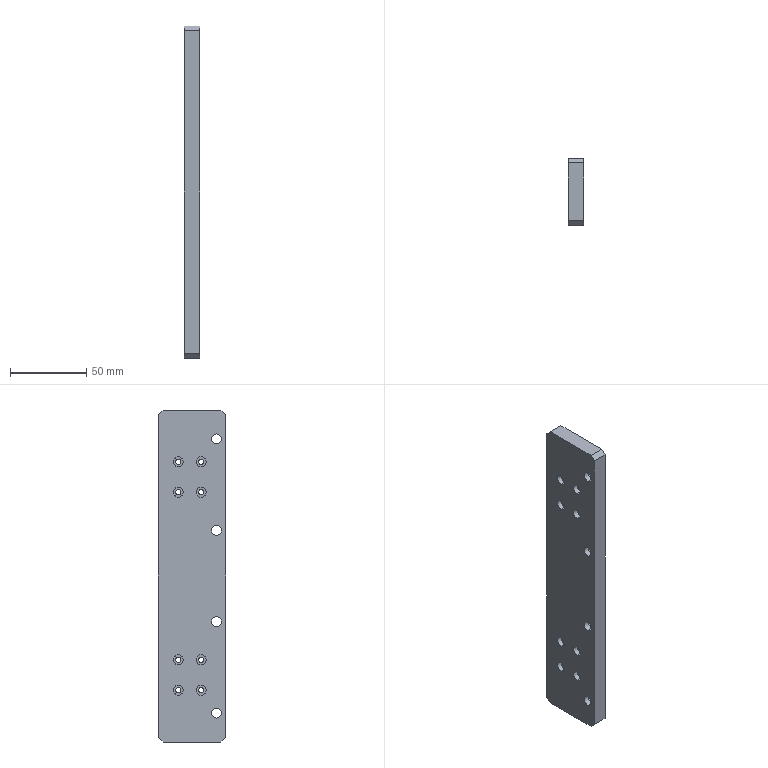Component | SolidWorks | 8TC-A15004-D0-11A-1 | 1 solid | 70 faces | box 10 x 44 x 218 mm | volume 91433 mm3 | cylinder 48 | plane 22 | commonest cylinder face diameters 6.5 x16 3.4 x16 11 x8 6.6 x8 | material #45
build123d program:
from build123d import *

# Parameters (mm, degrees)
SKETCH1_W                                       = 44
SKETCH1_H                                       = 218
BOSS_EXTRUDE1_DEPTH                             = 5
CHAMFER1_SIZE                                   = 3
M3_HEX_SOCKET_HEAD_CAP_SCREW_CBORE1_D           = 3.4
M3_HEX_SOCKET_HEAD_CAP_SCREW_CBORE1_CBORE_D     = 6.5
M3_HEX_SOCKET_HEAD_CAP_SCREW_CBORE1_CBORE_DEPTH = 3.4
M6_HEX_SOCKET_HEAD_CAP_SCREW_CBORE1_D           = 6.6
M6_HEX_SOCKET_HEAD_CAP_SCREW_CBORE1_CBORE_D     = 11
M6_HEX_SOCKET_HEAD_CAP_SCREW_CBORE1_CBORE_DEPTH = 6.4


with BuildPart() as part:
    # Sketch1 → Boss-Extrude1 (new, symmetric)
    with BuildSketch(Plane(origin=(0, 0, 0), x_dir=(1, 0, 0), z_dir=(0, 1, 0))):
        Rectangle(SKETCH1_W, SKETCH1_H)
    extrude(amount=BOSS_EXTRUDE1_DEPTH, both=True)

    # Chamfer1
    chamfer1_edges = [part.edges().sort_by_distance(p)[0] for p in [
        (22, 0, 109),
        (-22, 0, 109),
        (-22, 0, -109),
        (22, 0, -109),
    ]]
    chamfer(chamfer1_edges, length=CHAMFER1_SIZE)

    # M3 Hex Socket Head Cap Screw CBORE1 (through all)
    with Locations(Plane(origin=(0, 5, 0), x_dir=(1, 0, 0), z_dir=(0, 1, 0))):
        with Locations((-9, 75), (-9, 55), (6, 55), (6, 75), (6, -75), (6, -55), (-9, -55), (-9, -75)):
            CounterBoreHole(M3_HEX_SOCKET_HEAD_CAP_SCREW_CBORE1_D / 2, M3_HEX_SOCKET_HEAD_CAP_SCREW_CBORE1_CBORE_D / 2, M3_HEX_SOCKET_HEAD_CAP_SCREW_CBORE1_CBORE_DEPTH)

    # M6 Hex Socket Head Cap Screw CBORE1 (through all)
    with Locations(Plane(origin=(0, -5, 0), x_dir=(-1, 0, 0), z_dir=(0, -1, 0))):
        with Locations((-16, 90), (-16, 30), (-16, -30), (-16, -90)):
            CounterBoreHole(M6_HEX_SOCKET_HEAD_CAP_SCREW_CBORE1_D / 2, M6_HEX_SOCKET_HEAD_CAP_SCREW_CBORE1_CBORE_D / 2, M6_HEX_SOCKET_HEAD_CAP_SCREW_CBORE1_CBORE_DEPTH)


solid = part.part

# Placed as in the assembly
solid = solid.moved(Location((29.5, 354.5, 0), (180, 0, 90)))